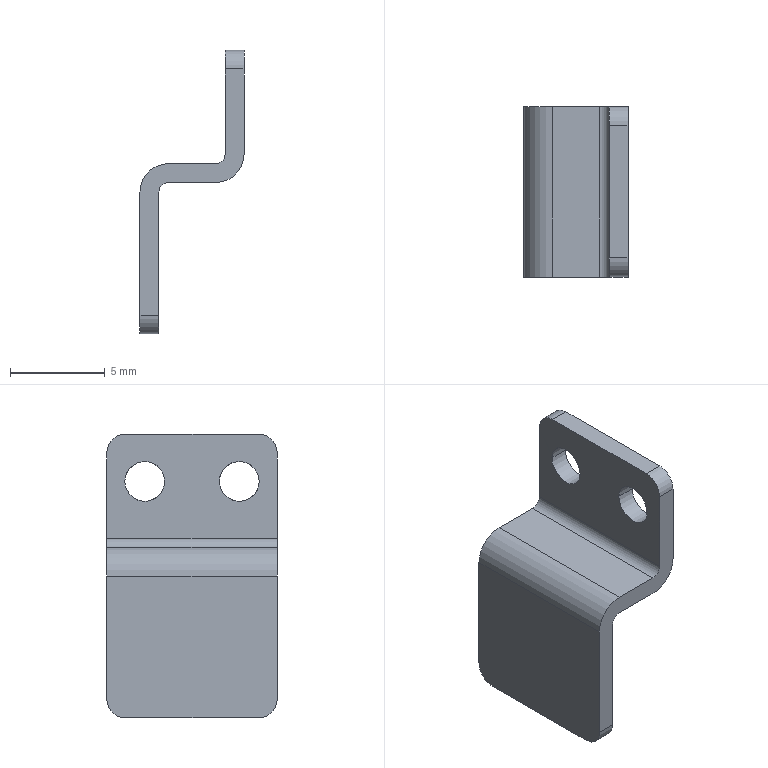Component | SolidWorks | 3359524133GTH5-400-BC(2)-1_GTH5-50-BC_slider2-1 | 1 solid | 22 faces | box 5.5 x 9 x 15 mm | volume 160 mm3 | cylinder 12 | plane 10 | commonest cylinder face diameters 2.1 x4 2 x4 3 x2 1 x2
STEP:
#1=COLOUR_RGB('',0.7922,0.8196,0.9333);
#2=FILL_AREA_STYLE_COLOUR('',#1);
#3=FILL_AREA_STYLE('',(#2));
#4=SURFACE_STYLE_FILL_AREA(#3);
#5=SURFACE_SIDE_STYLE('',(#4));
#6=SURFACE_STYLE_USAGE(.BOTH.,#5);
#7=PRESENTATION_STYLE_ASSIGNMENT((#6));
#8=CARTESIAN_POINT('',(13.183,43.162,-86.139));
#9=VERTEX_POINT('',#8);
#10=CARTESIAN_POINT('',(13.183,43.079,-86.139));
#11=VERTEX_POINT('',#10);
#12=CARTESIAN_POINT('',(13.183,43.162,-86.139));
#13=CARTESIAN_POINT('',(13.183,43.162,-86.145));
#14=CARTESIAN_POINT('',(13.183,43.161,-86.15));
#15=CARTESIAN_POINT('',(13.183,43.157,-86.16));
#16=CARTESIAN_POINT('',(13.183,43.154,-86.165));
#17=CARTESIAN_POINT('',(13.183,43.146,-86.172));
#18=CARTESIAN_POINT('',(13.183,43.142,-86.175));
#19=CARTESIAN_POINT('',(13.183,43.132,-86.179));
#20=CARTESIAN_POINT('',(13.183,43.126,-86.18));
#21=CARTESIAN_POINT('',(13.183,43.115,-86.18));
#22=CARTESIAN_POINT('',(13.183,43.11,-86.179));
#23=CARTESIAN_POINT('',(13.183,43.1,-86.175));
#24=CARTESIAN_POINT('',(13.183,43.095,-86.172));
#25=CARTESIAN_POINT('',(13.183,43.088,-86.165));
#26=CARTESIAN_POINT('',(13.183,43.085,-86.16));
#27=CARTESIAN_POINT('',(13.183,43.081,-86.15));
#28=CARTESIAN_POINT('',(13.183,43.079,-86.145));
#29=CARTESIAN_POINT('',(13.183,43.079,-86.139));
#30=B_SPLINE_CURVE_WITH_KNOTS('',3,(#12,#13,#14,#15,#16,#17,#18,#19,#20,#21,#22,#23,#24,#25,#26,#27,#28,#29),.UNSPECIFIED.,.F.,.F.,(4,2,2,2,2,2,2,2,4),(0.5,0.5625,0.625,0.6875,0.75,0.8125,0.875,0.9375,1.),.UNSPECIFIED.);
#31=EDGE_CURVE('',#9,#11,#30,.T.);
#32=ORIENTED_EDGE('',*,*,#31,.T.);
#33=CARTESIAN_POINT('',(13.222,43.079,-86.139));
#34=VERTEX_POINT('',#33);
#35=CARTESIAN_POINT('',(13.183,43.079,-86.139));
#36=DIRECTION('',(1.,0.,0.));
#37=VECTOR('',#36,39.37);
#38=LINE('',#35,#37);
#39=EDGE_CURVE('',#11,#34,#38,.T.);
#40=ORIENTED_EDGE('',*,*,#39,.T.);
#41=CARTESIAN_POINT('',(13.222,43.162,-86.139));
#42=VERTEX_POINT('',#41);
#43=CARTESIAN_POINT('',(13.222,43.121,-86.139));
#44=DIRECTION('',(1.,0.,0.));
#45=DIRECTION('',(0.,-1.,0.));
#46=AXIS2_PLACEMENT_3D('',#43,#44,#45);
#47=CIRCLE('',#46,0.04134);
#48=EDGE_CURVE('',#34,#42,#47,.T.);
#49=ORIENTED_EDGE('',*,*,#48,.T.);
#50=CARTESIAN_POINT('',(13.183,43.162,-86.139));
#51=DIRECTION('',(1.,0.,0.));
#52=VECTOR('',#51,39.37);
#53=LINE('',#50,#52);
#54=EDGE_CURVE('',#9,#42,#53,.T.);
#55=ORIENTED_EDGE('',*,*,#54,.F.);
#56=EDGE_LOOP('',(#32,#40,#49,#55));
#57=FACE_OUTER_BOUND('',#56,.T.);
#58=CARTESIAN_POINT('',(13.183,43.121,-86.139));
#59=DIRECTION('',(1.,0.,0.));
#60=DIRECTION('',(0.,1.,0.));
#61=AXIS2_PLACEMENT_3D('',#58,#59,#60);
#62=CYLINDRICAL_SURFACE('',#61,0.04134);
#63=ADVANCED_FACE('',(#57),#62,.F.);
#64=CARTESIAN_POINT('',(13.183,43.359,-86.139));
#65=VERTEX_POINT('',#64);
#66=CARTESIAN_POINT('',(13.183,43.276,-86.139));
#67=VERTEX_POINT('',#66);
#68=CARTESIAN_POINT('',(13.183,43.359,-86.139));
#69=CARTESIAN_POINT('',(13.183,43.359,-86.145));
#70=CARTESIAN_POINT('',(13.183,43.358,-86.15));
#71=CARTESIAN_POINT('',(13.183,43.354,-86.16));
#72=CARTESIAN_POINT('',(13.183,43.351,-86.165));
#73=CARTESIAN_POINT('',(13.183,43.343,-86.172));
#74=CARTESIAN_POINT('',(13.183,43.338,-86.175));
#75=CARTESIAN_POINT('',(13.183,43.328,-86.179));
#76=CARTESIAN_POINT('',(13.183,43.323,-86.18));
#77=CARTESIAN_POINT('',(13.183,43.312,-86.18));
#78=CARTESIAN_POINT('',(13.183,43.307,-86.179));
#79=CARTESIAN_POINT('',(13.183,43.297,-86.175));
#80=CARTESIAN_POINT('',(13.183,43.292,-86.172));
#81=CARTESIAN_POINT('',(13.183,43.285,-86.165));
#82=CARTESIAN_POINT('',(13.183,43.282,-86.16));
#83=CARTESIAN_POINT('',(13.183,43.277,-86.15));
#84=CARTESIAN_POINT('',(13.183,43.276,-86.145));
#85=CARTESIAN_POINT('',(13.183,43.276,-86.139));
#86=B_SPLINE_CURVE_WITH_KNOTS('',3,(#68,#69,#70,#71,#72,#73,#74,#75,#76,#77,#78,#79,#80,#81,#82,#83,#84,#85),.UNSPECIFIED.,.F.,.F.,(4,2,2,2,2,2,2,2,4),(0.5,0.5625,0.625,0.6875,0.75,0.8125,0.875,0.9375,1.),.UNSPECIFIED.);
#87=EDGE_CURVE('',#65,#67,#86,.T.);
#88=ORIENTED_EDGE('',*,*,#87,.T.);
#89=CARTESIAN_POINT('',(13.222,43.276,-86.139));
#90=VERTEX_POINT('',#89);
#91=CARTESIAN_POINT('',(13.183,43.276,-86.139));
#92=DIRECTION('',(1.,0.,0.));
#93=VECTOR('',#92,39.37);
#94=LINE('',#91,#93);
#95=EDGE_CURVE('',#67,#90,#94,.T.);
#96=ORIENTED_EDGE('',*,*,#95,.T.);
#97=CARTESIAN_POINT('',(13.222,43.359,-86.139));
#98=VERTEX_POINT('',#97);
#99=CARTESIAN_POINT('',(13.222,43.318,-86.139));
#100=DIRECTION('',(1.,0.,0.));
#101=DIRECTION('',(0.,-1.,0.));
#102=AXIS2_PLACEMENT_3D('',#99,#100,#101);
#103=CIRCLE('',#102,0.04134);
#104=EDGE_CURVE('',#90,#98,#103,.T.);
#105=ORIENTED_EDGE('',*,*,#104,.T.);
#106=CARTESIAN_POINT('',(13.183,43.359,-86.139));
#107=DIRECTION('',(1.,0.,0.));
#108=VECTOR('',#107,39.37);
#109=LINE('',#106,#108);
#110=EDGE_CURVE('',#65,#98,#109,.T.);
#111=ORIENTED_EDGE('',*,*,#110,.F.);
#112=EDGE_LOOP('',(#88,#96,#105,#111));
#113=FACE_OUTER_BOUND('',#112,.T.);
#114=CARTESIAN_POINT('',(13.183,43.318,-86.139));
#115=DIRECTION('',(1.,0.,0.));
#116=DIRECTION('',(0.,1.,0.));
#117=AXIS2_PLACEMENT_3D('',#114,#115,#116);
#118=CYLINDRICAL_SURFACE('',#117,0.04134);
#119=ADVANCED_FACE('',(#113),#118,.F.);
#120=CARTESIAN_POINT('',(13.183,43.081,-86.041));
#121=VERTEX_POINT('',#120);
#122=CARTESIAN_POINT('',(13.183,43.357,-86.041));
#123=VERTEX_POINT('',#122);
#124=CARTESIAN_POINT('',(13.183,43.042,-86.041));
#125=DIRECTION('',(0.,1.,0.));
#126=VECTOR('',#125,39.37);
#127=LINE('',#124,#126);
#128=EDGE_CURVE('',#121,#123,#127,.T.);
#129=ORIENTED_EDGE('',*,*,#128,.T.);
#130=CARTESIAN_POINT('',(13.183,43.396,-86.08));
#131=VERTEX_POINT('',#130);
#132=CARTESIAN_POINT('',(13.183,43.357,-86.08));
#133=DIRECTION('',(-1.,0.,0.));
#134=DIRECTION('',(0.,1.,0.));
#135=AXIS2_PLACEMENT_3D('',#132,#133,#134);
#136=CIRCLE('',#135,0.03937);
#137=EDGE_CURVE('',#123,#131,#136,.T.);
#138=ORIENTED_EDGE('',*,*,#137,.T.);
#139=CARTESIAN_POINT('',(13.183,43.396,-86.257));
#140=VERTEX_POINT('',#139);
#141=CARTESIAN_POINT('',(13.183,43.396,-86.041));
#142=DIRECTION('',(0.,-0.,-1.));
#143=VECTOR('',#142,39.37);
#144=LINE('',#141,#143);
#145=EDGE_CURVE('',#131,#140,#144,.T.);
#146=ORIENTED_EDGE('',*,*,#145,.T.);
#147=CARTESIAN_POINT('',(13.183,43.042,-86.257));
#148=VERTEX_POINT('',#147);
#149=CARTESIAN_POINT('',(13.183,43.042,-86.257));
#150=DIRECTION('',(0.,1.,0.));
#151=VECTOR('',#150,39.37);
#152=LINE('',#149,#151);
#153=EDGE_CURVE('',#148,#140,#152,.T.);
#154=ORIENTED_EDGE('',*,*,#153,.F.);
#155=CARTESIAN_POINT('',(13.183,43.042,-86.08));
#156=VERTEX_POINT('',#155);
#157=CARTESIAN_POINT('',(13.183,43.042,-86.041));
#158=DIRECTION('',(0.,-0.,-1.));
#159=VECTOR('',#158,39.37);
#160=LINE('',#157,#159);
#161=EDGE_CURVE('',#156,#148,#160,.T.);
#162=ORIENTED_EDGE('',*,*,#161,.F.);
#163=CARTESIAN_POINT('',(13.183,43.081,-86.08));
#164=DIRECTION('',(-1.,0.,0.));
#165=DIRECTION('',(0.,1.,0.));
#166=AXIS2_PLACEMENT_3D('',#163,#164,#165);
#167=CIRCLE('',#166,0.03937);
#168=EDGE_CURVE('',#156,#121,#167,.T.);
#169=ORIENTED_EDGE('',*,*,#168,.T.);
#170=EDGE_LOOP('',(#129,#138,#146,#154,#162,#169));
#171=FACE_OUTER_BOUND('',#170,.T.);
#172=ORIENTED_EDGE('',*,*,#87,.F.);
#173=CARTESIAN_POINT('',(13.183,43.276,-86.139));
#174=CARTESIAN_POINT('',(13.183,43.276,-86.134));
#175=CARTESIAN_POINT('',(13.183,43.277,-86.128));
#176=CARTESIAN_POINT('',(13.183,43.282,-86.118));
#177=CARTESIAN_POINT('',(13.183,43.285,-86.114));
#178=CARTESIAN_POINT('',(13.183,43.292,-86.106));
#179=CARTESIAN_POINT('',(13.183,43.297,-86.103));
#180=CARTESIAN_POINT('',(13.183,43.307,-86.099));
#181=CARTESIAN_POINT('',(13.183,43.312,-86.098));
#182=CARTESIAN_POINT('',(13.183,43.323,-86.098));
#183=CARTESIAN_POINT('',(13.183,43.328,-86.099));
#184=CARTESIAN_POINT('',(13.183,43.338,-86.103));
#185=CARTESIAN_POINT('',(13.183,43.343,-86.106));
#186=CARTESIAN_POINT('',(13.183,43.351,-86.114));
#187=CARTESIAN_POINT('',(13.183,43.354,-86.118));
#188=CARTESIAN_POINT('',(13.183,43.358,-86.128));
#189=CARTESIAN_POINT('',(13.183,43.359,-86.134));
#190=CARTESIAN_POINT('',(13.183,43.359,-86.139));
#191=B_SPLINE_CURVE_WITH_KNOTS('',3,(#173,#174,#175,#176,#177,#178,#179,#180,#181,#182,#183,#184,#185,#186,#187,#188,#189,#190),.UNSPECIFIED.,.F.,.F.,(4,2,2,2,2,2,2,2,4),(0.,0.0625,0.125,0.1875,0.25,0.3125,0.375,0.4375,0.5),.UNSPECIFIED.);
#192=EDGE_CURVE('',#67,#65,#191,.T.);
#193=ORIENTED_EDGE('',*,*,#192,.F.);
#194=EDGE_LOOP('',(#172,#193));
#195=FACE_BOUND('',#194,.T.);
#196=ORIENTED_EDGE('',*,*,#31,.F.);
#197=CARTESIAN_POINT('',(13.183,43.079,-86.139));
#198=CARTESIAN_POINT('',(13.183,43.079,-86.134));
#199=CARTESIAN_POINT('',(13.183,43.081,-86.128));
#200=CARTESIAN_POINT('',(13.183,43.085,-86.118));
#201=CARTESIAN_POINT('',(13.183,43.088,-86.114));
#202=CARTESIAN_POINT('',(13.183,43.095,-86.106));
#203=CARTESIAN_POINT('',(13.183,43.1,-86.103));
#204=CARTESIAN_POINT('',(13.183,43.11,-86.099));
#205=CARTESIAN_POINT('',(13.183,43.115,-86.098));
#206=CARTESIAN_POINT('',(13.183,43.126,-86.098));
#207=CARTESIAN_POINT('',(13.183,43.132,-86.099));
#208=CARTESIAN_POINT('',(13.183,43.142,-86.103));
#209=CARTESIAN_POINT('',(13.183,43.146,-86.106));
#210=CARTESIAN_POINT('',(13.183,43.154,-86.114));
#211=CARTESIAN_POINT('',(13.183,43.157,-86.118));
#212=CARTESIAN_POINT('',(13.183,43.161,-86.128));
#213=CARTESIAN_POINT('',(13.183,43.162,-86.134));
#214=CARTESIAN_POINT('',(13.183,43.162,-86.139));
#215=B_SPLINE_CURVE_WITH_KNOTS('',3,(#197,#198,#199,#200,#201,#202,#203,#204,#205,#206,#207,#208,#209,#210,#211,#212,#213,#214),.UNSPECIFIED.,.F.,.F.,(4,2,2,2,2,2,2,2,4),(0.,0.0625,0.125,0.1875,0.25,0.3125,0.375,0.4375,0.5),.UNSPECIFIED.);
#216=EDGE_CURVE('',#11,#9,#215,.T.);
#217=ORIENTED_EDGE('',*,*,#216,.F.);
#218=EDGE_LOOP('',(#196,#217));
#219=FACE_BOUND('',#218,.T.);
#220=CARTESIAN_POINT('',(13.183,43.042,-86.041));
#221=DIRECTION('',(1.,0.,0.));
#222=DIRECTION('',(0.,-0.,-1.));
#223=AXIS2_PLACEMENT_3D('',#220,#221,#222);
#224=PLANE('',#223);
#225=ADVANCED_FACE('',(#171,#195,#219),#224,.F.);
#226=CARTESIAN_POINT('',(13.006,43.081,-86.631));
#227=VERTEX_POINT('',#226);
#228=CARTESIAN_POINT('',(13.006,43.357,-86.631));
#229=VERTEX_POINT('',#228);
#230=CARTESIAN_POINT('',(13.006,43.042,-86.631));
#231=DIRECTION('',(0.,1.,0.));
#232=VECTOR('',#231,39.37);
#233=LINE('',#230,#232);
#234=EDGE_CURVE('',#227,#229,#233,.T.);
#235=ORIENTED_EDGE('',*,*,#234,.F.);
#236=CARTESIAN_POINT('',(13.006,43.042,-86.592));
#237=VERTEX_POINT('',#236);
#238=CARTESIAN_POINT('',(13.006,43.081,-86.592));
#239=DIRECTION('',(-1.,0.,0.));
#240=DIRECTION('',(0.,1.,0.));
#241=AXIS2_PLACEMENT_3D('',#238,#239,#240);
#242=CIRCLE('',#241,0.03937);
#243=EDGE_CURVE('',#227,#237,#242,.T.);
#244=ORIENTED_EDGE('',*,*,#243,.T.);
#245=CARTESIAN_POINT('',(13.006,43.042,-86.336));
#246=VERTEX_POINT('',#245);
#247=CARTESIAN_POINT('',(13.006,43.042,-86.336));
#248=DIRECTION('',(0.,-0.,-1.));
#249=VECTOR('',#248,39.37);
#250=LINE('',#247,#249);
#251=EDGE_CURVE('',#246,#237,#250,.T.);
#252=ORIENTED_EDGE('',*,*,#251,.F.);
#253=CARTESIAN_POINT('',(13.006,43.396,-86.336));
#254=VERTEX_POINT('',#253);
#255=CARTESIAN_POINT('',(13.006,43.042,-86.336));
#256=DIRECTION('',(0.,1.,0.));
#257=VECTOR('',#256,39.37);
#258=LINE('',#255,#257);
#259=EDGE_CURVE('',#246,#254,#258,.T.);
#260=ORIENTED_EDGE('',*,*,#259,.T.);
#261=CARTESIAN_POINT('',(13.006,43.396,-86.592));
#262=VERTEX_POINT('',#261);
#263=CARTESIAN_POINT('',(13.006,43.396,-86.336));
#264=DIRECTION('',(0.,-0.,-1.));
#265=VECTOR('',#264,39.37);
#266=LINE('',#263,#265);
#267=EDGE_CURVE('',#254,#262,#266,.T.);
#268=ORIENTED_EDGE('',*,*,#267,.T.);
#269=CARTESIAN_POINT('',(13.006,43.357,-86.592));
#270=DIRECTION('',(-1.,0.,0.));
#271=DIRECTION('',(0.,1.,0.));
#272=AXIS2_PLACEMENT_3D('',#269,#270,#271);
#273=CIRCLE('',#272,0.03937);
#274=EDGE_CURVE('',#262,#229,#273,.T.);
#275=ORIENTED_EDGE('',*,*,#274,.T.);
#276=EDGE_LOOP('',(#235,#244,#252,#260,#268,#275));
#277=FACE_OUTER_BOUND('',#276,.T.);
#278=CARTESIAN_POINT('',(13.006,43.042,-86.336));
#279=DIRECTION('',(1.,0.,0.));
#280=DIRECTION('',(0.,-0.,-1.));
#281=AXIS2_PLACEMENT_3D('',#278,#279,#280);
#282=PLANE('',#281);
#283=ADVANCED_FACE('',(#277),#282,.F.);
#284=CARTESIAN_POINT('',(13.222,43.357,-86.041));
#285=VERTEX_POINT('',#284);
#286=CARTESIAN_POINT('',(12.592,43.357,-86.041));
#287=DIRECTION('',(1.,0.,0.));
#288=VECTOR('',#287,39.37);
#289=LINE('',#286,#288);
#290=EDGE_CURVE('',#123,#285,#289,.T.);
#291=ORIENTED_EDGE('',*,*,#290,.T.);
#292=CARTESIAN_POINT('',(13.222,43.396,-86.08));
#293=VERTEX_POINT('',#292);
#294=CARTESIAN_POINT('',(13.222,43.357,-86.08));
#295=DIRECTION('',(-1.,0.,0.));
#296=DIRECTION('',(0.,-1.,0.));
#297=AXIS2_PLACEMENT_3D('',#294,#295,#296);
#298=CIRCLE('',#297,0.03937);
#299=EDGE_CURVE('',#285,#293,#298,.T.);
#300=ORIENTED_EDGE('',*,*,#299,.T.);
#301=CARTESIAN_POINT('',(12.592,43.396,-86.08));
#302=DIRECTION('',(-1.,0.,0.));
#303=VECTOR('',#302,39.37);
#304=LINE('',#301,#303);
#305=EDGE_CURVE('',#293,#131,#304,.T.);
#306=ORIENTED_EDGE('',*,*,#305,.T.);
#307=ORIENTED_EDGE('',*,*,#137,.F.);
#308=EDGE_LOOP('',(#291,#300,#306,#307));
#309=FACE_OUTER_BOUND('',#308,.T.);
#310=CARTESIAN_POINT('',(12.592,43.357,-86.08));
#311=DIRECTION('',(-1.,0.,0.));
#312=DIRECTION('',(0.,1.,0.));
#313=AXIS2_PLACEMENT_3D('',#310,#311,#312);
#314=CYLINDRICAL_SURFACE('',#313,0.03937);
#315=ADVANCED_FACE('',(#309),#314,.T.);
#316=CARTESIAN_POINT('',(13.222,43.042,-86.08));
#317=VERTEX_POINT('',#316);
#318=CARTESIAN_POINT('',(12.592,43.042,-86.08));
#319=DIRECTION('',(-1.,0.,0.));
#320=VECTOR('',#319,39.37);
#321=LINE('',#318,#320);
#322=EDGE_CURVE('',#317,#156,#321,.T.);
#323=ORIENTED_EDGE('',*,*,#322,.F.);
#324=CARTESIAN_POINT('',(13.222,43.081,-86.041));
#325=VERTEX_POINT('',#324);
#326=CARTESIAN_POINT('',(13.222,43.081,-86.08));
#327=DIRECTION('',(-1.,0.,0.));
#328=DIRECTION('',(0.,-1.,0.));
#329=AXIS2_PLACEMENT_3D('',#326,#327,#328);
#330=CIRCLE('',#329,0.03937);
#331=EDGE_CURVE('',#317,#325,#330,.T.);
#332=ORIENTED_EDGE('',*,*,#331,.T.);
#333=CARTESIAN_POINT('',(12.592,43.081,-86.041));
#334=DIRECTION('',(1.,0.,0.));
#335=VECTOR('',#334,39.37);
#336=LINE('',#333,#335);
#337=EDGE_CURVE('',#121,#325,#336,.T.);
#338=ORIENTED_EDGE('',*,*,#337,.F.);
#339=ORIENTED_EDGE('',*,*,#168,.F.);
#340=EDGE_LOOP('',(#323,#332,#338,#339));
#341=FACE_OUTER_BOUND('',#340,.T.);
#342=CARTESIAN_POINT('',(12.592,43.081,-86.08));
#343=DIRECTION('',(-1.,0.,0.));
#344=DIRECTION('',(0.,1.,0.));
#345=AXIS2_PLACEMENT_3D('',#342,#343,#344);
#346=CYLINDRICAL_SURFACE('',#345,0.03937);
#347=ADVANCED_FACE('',(#341),#346,.T.);
#348=CARTESIAN_POINT('',(13.045,43.081,-86.631));
#349=VERTEX_POINT('',#348);
#350=CARTESIAN_POINT('',(12.592,43.081,-86.631));
#351=DIRECTION('',(1.,0.,0.));
#352=VECTOR('',#351,39.37);
#353=LINE('',#350,#352);
#354=EDGE_CURVE('',#227,#349,#353,.T.);
#355=ORIENTED_EDGE('',*,*,#354,.T.);
#356=CARTESIAN_POINT('',(13.045,43.042,-86.592));
#357=VERTEX_POINT('',#356);
#358=CARTESIAN_POINT('',(13.045,43.081,-86.592));
#359=DIRECTION('',(1.,0.,0.));
#360=DIRECTION('',(0.,-1.,0.));
#361=AXIS2_PLACEMENT_3D('',#358,#359,#360);
#362=CIRCLE('',#361,0.03937);
#363=EDGE_CURVE('',#357,#349,#362,.T.);
#364=ORIENTED_EDGE('',*,*,#363,.F.);
#365=CARTESIAN_POINT('',(12.592,43.042,-86.592));
#366=DIRECTION('',(-1.,0.,0.));
#367=VECTOR('',#366,39.37);
#368=LINE('',#365,#367);
#369=EDGE_CURVE('',#357,#237,#368,.T.);
#370=ORIENTED_EDGE('',*,*,#369,.T.);
#371=ORIENTED_EDGE('',*,*,#243,.F.);
#372=EDGE_LOOP('',(#355,#364,#370,#371));
#373=FACE_OUTER_BOUND('',#372,.T.);
#374=CARTESIAN_POINT('',(12.592,43.081,-86.592));
#375=DIRECTION('',(-1.,0.,0.));
#376=DIRECTION('',(0.,1.,0.));
#377=AXIS2_PLACEMENT_3D('',#374,#375,#376);
#378=CYLINDRICAL_SURFACE('',#377,0.03937);
#379=ADVANCED_FACE('',(#373),#378,.T.);
#380=CARTESIAN_POINT('',(13.045,43.396,-86.592));
#381=VERTEX_POINT('',#380);
#382=CARTESIAN_POINT('',(12.592,43.396,-86.592));
#383=DIRECTION('',(-1.,0.,0.));
#384=VECTOR('',#383,39.37);
#385=LINE('',#382,#384);
#386=EDGE_CURVE('',#381,#262,#385,.T.);
#387=ORIENTED_EDGE('',*,*,#386,.F.);
#388=CARTESIAN_POINT('',(13.045,43.357,-86.631));
#389=VERTEX_POINT('',#388);
#390=CARTESIAN_POINT('',(13.045,43.357,-86.592));
#391=DIRECTION('',(1.,0.,0.));
#392=DIRECTION('',(0.,-1.,0.));
#393=AXIS2_PLACEMENT_3D('',#390,#391,#392);
#394=CIRCLE('',#393,0.03937);
#395=EDGE_CURVE('',#389,#381,#394,.T.);
#396=ORIENTED_EDGE('',*,*,#395,.F.);
#397=CARTESIAN_POINT('',(12.592,43.357,-86.631));
#398=DIRECTION('',(1.,0.,0.));
#399=VECTOR('',#398,39.37);
#400=LINE('',#397,#399);
#401=EDGE_CURVE('',#229,#389,#400,.T.);
#402=ORIENTED_EDGE('',*,*,#401,.F.);
#403=ORIENTED_EDGE('',*,*,#274,.F.);
#404=EDGE_LOOP('',(#387,#396,#402,#403));
#405=FACE_OUTER_BOUND('',#404,.T.);
#406=CARTESIAN_POINT('',(12.592,43.357,-86.592));
#407=DIRECTION('',(-1.,0.,0.));
#408=DIRECTION('',(0.,1.,0.));
#409=AXIS2_PLACEMENT_3D('',#406,#407,#408);
#410=CYLINDRICAL_SURFACE('',#409,0.03937);
#411=ADVANCED_FACE('',(#405),#410,.T.);
#412=CARTESIAN_POINT('',(13.222,43.042,-86.257));
#413=VERTEX_POINT('',#412);
#414=CARTESIAN_POINT('',(13.222,43.042,-86.257));
#415=DIRECTION('',(0.,0.,1.));
#416=VECTOR('',#415,39.37);
#417=LINE('',#414,#416);
#418=EDGE_CURVE('',#413,#317,#417,.T.);
#419=ORIENTED_EDGE('',*,*,#418,.T.);
#420=ORIENTED_EDGE('',*,*,#322,.T.);
#421=ORIENTED_EDGE('',*,*,#161,.T.);
#422=CARTESIAN_POINT('',(13.163,43.042,-86.277));
#423=VERTEX_POINT('',#422);
#424=CARTESIAN_POINT('',(13.163,43.042,-86.257));
#425=DIRECTION('',(0.,-1.,-0.));
#426=DIRECTION('',(1.,0.,0.));
#427=AXIS2_PLACEMENT_3D('',#424,#425,#426);
#428=CIRCLE('',#427,0.01969);
#429=EDGE_CURVE('',#423,#148,#428,.T.);
#430=ORIENTED_EDGE('',*,*,#429,.F.);
#431=CARTESIAN_POINT('',(13.065,43.042,-86.277));
#432=VERTEX_POINT('',#431);
#433=CARTESIAN_POINT('',(13.163,43.042,-86.277));
#434=DIRECTION('',(-1.,0.,0.));
#435=VECTOR('',#434,39.37);
#436=LINE('',#433,#435);
#437=EDGE_CURVE('',#423,#432,#436,.T.);
#438=ORIENTED_EDGE('',*,*,#437,.T.);
#439=CARTESIAN_POINT('',(13.065,43.042,-86.336));
#440=DIRECTION('',(0.,-1.,-0.));
#441=DIRECTION('',(1.,0.,0.));
#442=AXIS2_PLACEMENT_3D('',#439,#440,#441);
#443=CIRCLE('',#442,0.05906);
#444=EDGE_CURVE('',#432,#246,#443,.T.);
#445=ORIENTED_EDGE('',*,*,#444,.T.);
#446=ORIENTED_EDGE('',*,*,#251,.T.);
#447=ORIENTED_EDGE('',*,*,#369,.F.);
#448=CARTESIAN_POINT('',(13.045,43.042,-86.336));
#449=VERTEX_POINT('',#448);
#450=CARTESIAN_POINT('',(13.045,43.042,-86.631));
#451=DIRECTION('',(0.,0.,1.));
#452=VECTOR('',#451,39.37);
#453=LINE('',#450,#452);
#454=EDGE_CURVE('',#357,#449,#453,.T.);
#455=ORIENTED_EDGE('',*,*,#454,.T.);
#456=CARTESIAN_POINT('',(13.065,43.042,-86.316));
#457=VERTEX_POINT('',#456);
#458=CARTESIAN_POINT('',(13.065,43.042,-86.336));
#459=DIRECTION('',(0.,-1.,-0.));
#460=DIRECTION('',(1.,0.,0.));
#461=AXIS2_PLACEMENT_3D('',#458,#459,#460);
#462=CIRCLE('',#461,0.01969);
#463=EDGE_CURVE('',#457,#449,#462,.T.);
#464=ORIENTED_EDGE('',*,*,#463,.F.);
#465=CARTESIAN_POINT('',(13.163,43.042,-86.316));
#466=VERTEX_POINT('',#465);
#467=CARTESIAN_POINT('',(13.065,43.042,-86.316));
#468=DIRECTION('',(1.,0.,0.));
#469=VECTOR('',#468,39.37);
#470=LINE('',#467,#469);
#471=EDGE_CURVE('',#457,#466,#470,.T.);
#472=ORIENTED_EDGE('',*,*,#471,.T.);
#473=CARTESIAN_POINT('',(13.163,43.042,-86.257));
#474=DIRECTION('',(0.,-1.,-0.));
#475=DIRECTION('',(1.,0.,0.));
#476=AXIS2_PLACEMENT_3D('',#473,#474,#475);
#477=CIRCLE('',#476,0.05906);
#478=EDGE_CURVE('',#466,#413,#477,.T.);
#479=ORIENTED_EDGE('',*,*,#478,.T.);
#480=EDGE_LOOP('',(#419,#420,#421,#430,#438,#445,#446,#447,#455,#464,#472,#479));
#481=FACE_OUTER_BOUND('',#480,.T.);
#482=CARTESIAN_POINT('',(13.065,43.042,-86.336));
#483=DIRECTION('',(0.,-1.,0.));
#484=DIRECTION('',(0.,0.,1.));
#485=AXIS2_PLACEMENT_3D('',#482,#483,#484);
#486=PLANE('',#485);
#487=ADVANCED_FACE('',(#481),#486,.T.);
#488=ORIENTED_EDGE('',*,*,#305,.F.);
#489=CARTESIAN_POINT('',(13.222,43.396,-86.257));
#490=VERTEX_POINT('',#489);
#491=CARTESIAN_POINT('',(13.222,43.396,-86.257));
#492=DIRECTION('',(0.,0.,1.));
#493=VECTOR('',#492,39.37);
#494=LINE('',#491,#493);
#495=EDGE_CURVE('',#490,#293,#494,.T.);
#496=ORIENTED_EDGE('',*,*,#495,.F.);
#497=CARTESIAN_POINT('',(13.163,43.396,-86.316));
#498=VERTEX_POINT('',#497);
#499=CARTESIAN_POINT('',(13.163,43.396,-86.257));
#500=DIRECTION('',(0.,-1.,-0.));
#501=DIRECTION('',(1.,0.,0.));
#502=AXIS2_PLACEMENT_3D('',#499,#500,#501);
#503=CIRCLE('',#502,0.05906);
#504=EDGE_CURVE('',#498,#490,#503,.T.);
#505=ORIENTED_EDGE('',*,*,#504,.F.);
#506=CARTESIAN_POINT('',(13.065,43.396,-86.316));
#507=VERTEX_POINT('',#506);
#508=CARTESIAN_POINT('',(13.065,43.396,-86.316));
#509=DIRECTION('',(1.,0.,0.));
#510=VECTOR('',#509,39.37);
#511=LINE('',#508,#510);
#512=EDGE_CURVE('',#507,#498,#511,.T.);
#513=ORIENTED_EDGE('',*,*,#512,.F.);
#514=CARTESIAN_POINT('',(13.045,43.396,-86.336));
#515=VERTEX_POINT('',#514);
#516=CARTESIAN_POINT('',(13.065,43.396,-86.336));
#517=DIRECTION('',(0.,-1.,-0.));
#518=DIRECTION('',(1.,0.,0.));
#519=AXIS2_PLACEMENT_3D('',#516,#517,#518);
#520=CIRCLE('',#519,0.01969);
#521=EDGE_CURVE('',#507,#515,#520,.T.);
#522=ORIENTED_EDGE('',*,*,#521,.T.);
#523=CARTESIAN_POINT('',(13.045,43.396,-86.631));
#524=DIRECTION('',(0.,0.,1.));
#525=VECTOR('',#524,39.37);
#526=LINE('',#523,#525);
#527=EDGE_CURVE('',#381,#515,#526,.T.);
#528=ORIENTED_EDGE('',*,*,#527,.F.);
#529=ORIENTED_EDGE('',*,*,#386,.T.);
#530=ORIENTED_EDGE('',*,*,#267,.F.);
#531=CARTESIAN_POINT('',(13.065,43.396,-86.277));
#532=VERTEX_POINT('',#531);
#533=CARTESIAN_POINT('',(13.065,43.396,-86.336));
#534=DIRECTION('',(0.,-1.,-0.));
#535=DIRECTION('',(1.,0.,0.));
#536=AXIS2_PLACEMENT_3D('',#533,#534,#535);
#537=CIRCLE('',#536,0.05906);
#538=EDGE_CURVE('',#532,#254,#537,.T.);
#539=ORIENTED_EDGE('',*,*,#538,.F.);
#540=CARTESIAN_POINT('',(13.163,43.396,-86.277));
#541=VERTEX_POINT('',#540);
#542=CARTESIAN_POINT('',(13.163,43.396,-86.277));
#543=DIRECTION('',(-1.,0.,0.));
#544=VECTOR('',#543,39.37);
#545=LINE('',#542,#544);
#546=EDGE_CURVE('',#541,#532,#545,.T.);
#547=ORIENTED_EDGE('',*,*,#546,.F.);
#548=CARTESIAN_POINT('',(13.163,43.396,-86.257));
#549=DIRECTION('',(0.,-1.,-0.));
#550=DIRECTION('',(1.,0.,0.));
#551=AXIS2_PLACEMENT_3D('',#548,#549,#550);
#552=CIRCLE('',#551,0.01969);
#553=EDGE_CURVE('',#541,#140,#552,.T.);
#554=ORIENTED_EDGE('',*,*,#553,.T.);
#555=ORIENTED_EDGE('',*,*,#145,.F.);
#556=EDGE_LOOP('',(#488,#496,#505,#513,#522,#528,#529,#530,#539,#547,#554,#555));
#557=FACE_OUTER_BOUND('',#556,.T.);
#558=CARTESIAN_POINT('',(13.065,43.396,-86.336));
#559=DIRECTION('',(0.,-1.,0.));
#560=DIRECTION('',(0.,0.,1.));
#561=AXIS2_PLACEMENT_3D('',#558,#559,#560);
#562=PLANE('',#561);
#563=ADVANCED_FACE('',(#557),#562,.F.);
#564=ORIENTED_EDGE('',*,*,#538,.T.);
#565=ORIENTED_EDGE('',*,*,#259,.F.);
#566=ORIENTED_EDGE('',*,*,#444,.F.);
#567=CARTESIAN_POINT('',(13.065,43.042,-86.277));
#568=DIRECTION('',(0.,1.,0.));
#569=VECTOR('',#568,39.37);
#570=LINE('',#567,#569);
#571=EDGE_CURVE('',#432,#532,#570,.T.);
#572=ORIENTED_EDGE('',*,*,#571,.T.);
#573=EDGE_LOOP('',(#564,#565,#566,#572));
#574=FACE_OUTER_BOUND('',#573,.T.);
#575=CARTESIAN_POINT('',(13.065,43.042,-86.336));
#576=DIRECTION('',(0.,-1.,-0.));
#577=DIRECTION('',(-1.,0.,0.));
#578=AXIS2_PLACEMENT_3D('',#575,#576,#577);
#579=CYLINDRICAL_SURFACE('',#578,0.05906);
#580=ADVANCED_FACE('',(#574),#579,.T.);
#581=ORIENTED_EDGE('',*,*,#546,.T.);
#582=ORIENTED_EDGE('',*,*,#571,.F.);
#583=ORIENTED_EDGE('',*,*,#437,.F.);
#584=CARTESIAN_POINT('',(13.163,43.042,-86.277));
#585=DIRECTION('',(0.,1.,0.));
#586=VECTOR('',#585,39.37);
#587=LINE('',#584,#586);
#588=EDGE_CURVE('',#423,#541,#587,.T.);
#589=ORIENTED_EDGE('',*,*,#588,.T.);
#590=EDGE_LOOP('',(#581,#582,#583,#589));
#591=FACE_OUTER_BOUND('',#590,.T.);
#592=CARTESIAN_POINT('',(13.163,43.042,-86.277));
#593=DIRECTION('',(0.,-0.,-1.));
#594=DIRECTION('',(1.,0.,0.));
#595=AXIS2_PLACEMENT_3D('',#592,#593,#594);
#596=PLANE('',#595);
#597=ADVANCED_FACE('',(#591),#596,.F.);
#598=ORIENTED_EDGE('',*,*,#553,.F.);
#599=ORIENTED_EDGE('',*,*,#588,.F.);
#600=ORIENTED_EDGE('',*,*,#429,.T.);
#601=ORIENTED_EDGE('',*,*,#153,.T.);
#602=EDGE_LOOP('',(#598,#599,#600,#601));
#603=FACE_OUTER_BOUND('',#602,.T.);
#604=CARTESIAN_POINT('',(13.163,43.042,-86.257));
#605=DIRECTION('',(0.,-1.,-0.));
#606=DIRECTION('',(-1.,0.,0.));
#607=AXIS2_PLACEMENT_3D('',#604,#605,#606);
#608=CYLINDRICAL_SURFACE('',#607,0.01969);
#609=ADVANCED_FACE('',(#603),#608,.F.);
#610=CARTESIAN_POINT('',(13.222,43.121,-86.139));
#611=DIRECTION('',(1.,0.,0.));
#612=DIRECTION('',(0.,-1.,0.));
#613=AXIS2_PLACEMENT_3D('',#610,#611,#612);
#614=CIRCLE('',#613,0.04134);
#615=EDGE_CURVE('',#42,#34,#614,.T.);
#616=ORIENTED_EDGE('',*,*,#615,.F.);
#617=ORIENTED_EDGE('',*,*,#48,.F.);
#618=EDGE_LOOP('',(#616,#617));
#619=FACE_BOUND('',#618,.T.);
#620=CARTESIAN_POINT('',(13.222,43.318,-86.139));
#621=DIRECTION('',(1.,0.,0.));
#622=DIRECTION('',(0.,-1.,0.));
#623=AXIS2_PLACEMENT_3D('',#620,#621,#622);
#624=CIRCLE('',#623,0.04134);
#625=EDGE_CURVE('',#98,#90,#624,.T.);
#626=ORIENTED_EDGE('',*,*,#625,.F.);
#627=ORIENTED_EDGE('',*,*,#104,.F.);
#628=EDGE_LOOP('',(#626,#627));
#629=FACE_BOUND('',#628,.T.);
#630=ORIENTED_EDGE('',*,*,#495,.T.);
#631=ORIENTED_EDGE('',*,*,#299,.F.);
#632=CARTESIAN_POINT('',(13.222,43.042,-86.041));
#633=DIRECTION('',(0.,1.,0.));
#634=VECTOR('',#633,39.37);
#635=LINE('',#632,#634);
#636=EDGE_CURVE('',#325,#285,#635,.T.);
#637=ORIENTED_EDGE('',*,*,#636,.F.);
#638=ORIENTED_EDGE('',*,*,#331,.F.);
#639=ORIENTED_EDGE('',*,*,#418,.F.);
#640=CARTESIAN_POINT('',(13.222,43.042,-86.257));
#641=DIRECTION('',(0.,1.,0.));
#642=VECTOR('',#641,39.37);
#643=LINE('',#640,#642);
#644=EDGE_CURVE('',#413,#490,#643,.T.);
#645=ORIENTED_EDGE('',*,*,#644,.T.);
#646=EDGE_LOOP('',(#630,#631,#637,#638,#639,#645));
#647=FACE_OUTER_BOUND('',#646,.T.);
#648=CARTESIAN_POINT('',(13.222,43.042,-86.257));
#649=DIRECTION('',(-1.,0.,0.));
#650=DIRECTION('',(0.,-1.,-0.));
#651=AXIS2_PLACEMENT_3D('',#648,#649,#650);
#652=PLANE('',#651);
#653=ADVANCED_FACE('',(#619,#629,#647),#652,.F.);
#654=ORIENTED_EDGE('',*,*,#504,.T.);
#655=ORIENTED_EDGE('',*,*,#644,.F.);
#656=ORIENTED_EDGE('',*,*,#478,.F.);
#657=CARTESIAN_POINT('',(13.163,43.042,-86.316));
#658=DIRECTION('',(0.,1.,0.));
#659=VECTOR('',#658,39.37);
#660=LINE('',#657,#659);
#661=EDGE_CURVE('',#466,#498,#660,.T.);
#662=ORIENTED_EDGE('',*,*,#661,.T.);
#663=EDGE_LOOP('',(#654,#655,#656,#662));
#664=FACE_OUTER_BOUND('',#663,.T.);
#665=CARTESIAN_POINT('',(13.163,43.042,-86.257));
#666=DIRECTION('',(0.,-1.,-0.));
#667=DIRECTION('',(-1.,0.,0.));
#668=AXIS2_PLACEMENT_3D('',#665,#666,#667);
#669=CYLINDRICAL_SURFACE('',#668,0.05906);
#670=ADVANCED_FACE('',(#664),#669,.T.);
#671=ORIENTED_EDGE('',*,*,#512,.T.);
#672=ORIENTED_EDGE('',*,*,#661,.F.);
#673=ORIENTED_EDGE('',*,*,#471,.F.);
#674=CARTESIAN_POINT('',(13.065,43.042,-86.316));
#675=DIRECTION('',(0.,1.,0.));
#676=VECTOR('',#675,39.37);
#677=LINE('',#674,#676);
#678=EDGE_CURVE('',#457,#507,#677,.T.);
#679=ORIENTED_EDGE('',*,*,#678,.T.);
#680=EDGE_LOOP('',(#671,#672,#673,#679));
#681=FACE_OUTER_BOUND('',#680,.T.);
#682=CARTESIAN_POINT('',(13.065,43.042,-86.316));
#683=DIRECTION('',(0.,-0.,1.));
#684=DIRECTION('',(0.,-1.,-0.));
#685=AXIS2_PLACEMENT_3D('',#682,#683,#684);
#686=PLANE('',#685);
#687=ADVANCED_FACE('',(#681),#686,.F.);
#688=ORIENTED_EDGE('',*,*,#521,.F.);
#689=ORIENTED_EDGE('',*,*,#678,.F.);
#690=ORIENTED_EDGE('',*,*,#463,.T.);
#691=CARTESIAN_POINT('',(13.045,43.042,-86.336));
#692=DIRECTION('',(0.,1.,0.));
#693=VECTOR('',#692,39.37);
#694=LINE('',#691,#693);
#695=EDGE_CURVE('',#449,#515,#694,.T.);
#696=ORIENTED_EDGE('',*,*,#695,.T.);
#697=EDGE_LOOP('',(#688,#689,#690,#696));
#698=FACE_OUTER_BOUND('',#697,.T.);
#699=CARTESIAN_POINT('',(13.065,43.042,-86.336));
#700=DIRECTION('',(0.,-1.,-0.));
#701=DIRECTION('',(-1.,0.,0.));
#702=AXIS2_PLACEMENT_3D('',#699,#700,#701);
#703=CYLINDRICAL_SURFACE('',#702,0.01969);
#704=ADVANCED_FACE('',(#698),#703,.F.);
#705=ORIENTED_EDGE('',*,*,#454,.F.);
#706=ORIENTED_EDGE('',*,*,#363,.T.);
#707=CARTESIAN_POINT('',(13.045,43.042,-86.631));
#708=DIRECTION('',(0.,1.,0.));
#709=VECTOR('',#708,39.37);
#710=LINE('',#707,#709);
#711=EDGE_CURVE('',#349,#389,#710,.T.);
#712=ORIENTED_EDGE('',*,*,#711,.T.);
#713=ORIENTED_EDGE('',*,*,#395,.T.);
#714=ORIENTED_EDGE('',*,*,#527,.T.);
#715=ORIENTED_EDGE('',*,*,#695,.F.);
#716=EDGE_LOOP('',(#705,#706,#712,#713,#714,#715));
#717=FACE_OUTER_BOUND('',#716,.T.);
#718=CARTESIAN_POINT('',(13.045,43.042,-86.631));
#719=DIRECTION('',(-1.,0.,0.));
#720=DIRECTION('',(0.,-1.,-0.));
#721=AXIS2_PLACEMENT_3D('',#718,#719,#720);
#722=PLANE('',#721);
#723=ADVANCED_FACE('',(#717),#722,.F.);
#724=ORIENTED_EDGE('',*,*,#636,.T.);
#725=ORIENTED_EDGE('',*,*,#290,.F.);
#726=ORIENTED_EDGE('',*,*,#128,.F.);
#727=ORIENTED_EDGE('',*,*,#337,.T.);
#728=EDGE_LOOP('',(#724,#725,#726,#727));
#729=FACE_OUTER_BOUND('',#728,.T.);
#730=CARTESIAN_POINT('',(13.222,43.042,-86.041));
#731=DIRECTION('',(0.,-0.,-1.));
#732=DIRECTION('',(1.,0.,0.));
#733=AXIS2_PLACEMENT_3D('',#730,#731,#732);
#734=PLANE('',#733);
#735=ADVANCED_FACE('',(#729),#734,.F.);
#736=ORIENTED_EDGE('',*,*,#711,.F.);
#737=ORIENTED_EDGE('',*,*,#354,.F.);
#738=ORIENTED_EDGE('',*,*,#234,.T.);
#739=ORIENTED_EDGE('',*,*,#401,.T.);
#740=EDGE_LOOP('',(#736,#737,#738,#739));
#741=FACE_OUTER_BOUND('',#740,.T.);
#742=CARTESIAN_POINT('',(13.006,43.042,-86.631));
#743=DIRECTION('',(0.,-0.,1.));
#744=DIRECTION('',(0.,-1.,-0.));
#745=AXIS2_PLACEMENT_3D('',#742,#743,#744);
#746=PLANE('',#745);
#747=ADVANCED_FACE('',(#741),#746,.F.);
#748=ORIENTED_EDGE('',*,*,#95,.F.);
#749=ORIENTED_EDGE('',*,*,#192,.T.);
#750=ORIENTED_EDGE('',*,*,#110,.T.);
#751=ORIENTED_EDGE('',*,*,#625,.T.);
#752=EDGE_LOOP('',(#748,#749,#750,#751));
#753=FACE_OUTER_BOUND('',#752,.T.);
#754=CARTESIAN_POINT('',(13.183,43.318,-86.139));
#755=DIRECTION('',(1.,0.,0.));
#756=DIRECTION('',(0.,1.,0.));
#757=AXIS2_PLACEMENT_3D('',#754,#755,#756);
#758=CYLINDRICAL_SURFACE('',#757,0.04134);
#759=ADVANCED_FACE('',(#753),#758,.F.);
#760=ORIENTED_EDGE('',*,*,#39,.F.);
#761=ORIENTED_EDGE('',*,*,#216,.T.);
#762=ORIENTED_EDGE('',*,*,#54,.T.);
#763=ORIENTED_EDGE('',*,*,#615,.T.);
#764=EDGE_LOOP('',(#760,#761,#762,#763));
#765=FACE_OUTER_BOUND('',#764,.T.);
#766=CARTESIAN_POINT('',(13.183,43.121,-86.139));
#767=DIRECTION('',(1.,0.,0.));
#768=DIRECTION('',(0.,1.,0.));
#769=AXIS2_PLACEMENT_3D('',#766,#767,#768);
#770=CYLINDRICAL_SURFACE('',#769,0.04134);
#771=ADVANCED_FACE('',(#765),#770,.F.);
#772=CLOSED_SHELL('',(#63,#119,#225,#283,#315,#347,#379,#411,#487,#563,#580,#597,#609,#653,#670,#687,#704,#723,#735,#747,#759,#771));
#773=MANIFOLD_SOLID_BREP('',#772);
#774=STYLED_ITEM('',(#7),#773);
#775=PRESENTATION_LAYER_ASSIGNMENT('','',(#774));
#776=CARTESIAN_POINT('',(0.,0.,0.));
#777=DIRECTION('',(0.,0.,1.));
#778=DIRECTION('',(1.,0.,0.));
#779=AXIS2_PLACEMENT_3D('',#776,#777,#778);
#780=(LENGTH_UNIT()NAMED_UNIT(*)SI_UNIT($,.METRE.));
#781=LENGTH_MEASURE_WITH_UNIT(LENGTH_MEASURE(0.0254),#780);
#782=DIMENSIONAL_EXPONENTS(1.,0.,0.,0.,0.,0.,0.);
#783=(CONVERSION_BASED_UNIT('',#781)LENGTH_UNIT()NAMED_UNIT(#782));
#784=UNCERTAINTY_MEASURE_WITH_UNIT(LENGTH_MEASURE(0.00001),#783,'','');
#785=(NAMED_UNIT(*)PLANE_ANGLE_UNIT()SI_UNIT($,.RADIAN.));
#786=(NAMED_UNIT(*)SI_UNIT($,.STERADIAN.)SOLID_ANGLE_UNIT());
#787=(GEOMETRIC_REPRESENTATION_CONTEXT(3)GLOBAL_UNCERTAINTY_ASSIGNED_CONTEXT((#784))GLOBAL_UNIT_ASSIGNED_CONTEXT((#783,#785,#786))REPRESENTATION_CONTEXT('',''));
#788=ADVANCED_BREP_SHAPE_REPRESENTATION('',(#773,#779),#787);
#789=(LENGTH_UNIT()NAMED_UNIT(*)SI_UNIT($,.METRE.));
#790=LENGTH_MEASURE_WITH_UNIT(LENGTH_MEASURE(0.0254),#789);
#791=DIMENSIONAL_EXPONENTS(1.,0.,0.,0.,0.,0.,0.);
#792=(CONVERSION_BASED_UNIT('',#790)LENGTH_UNIT()NAMED_UNIT(#791));
#793=UNCERTAINTY_MEASURE_WITH_UNIT(LENGTH_MEASURE(0.00001),#792,'','');
#794=(NAMED_UNIT(*)PLANE_ANGLE_UNIT()SI_UNIT($,.RADIAN.));
#795=(NAMED_UNIT(*)SI_UNIT($,.STERADIAN.)SOLID_ANGLE_UNIT());
#796=(GEOMETRIC_REPRESENTATION_CONTEXT(3)GLOBAL_UNCERTAINTY_ASSIGNED_CONTEXT((#793))GLOBAL_UNIT_ASSIGNED_CONTEXT((#792,#794,#795))REPRESENTATION_CONTEXT('',''));
#797=MECHANICAL_DESIGN_GEOMETRIC_PRESENTATION_REPRESENTATION('',(#774),#796);